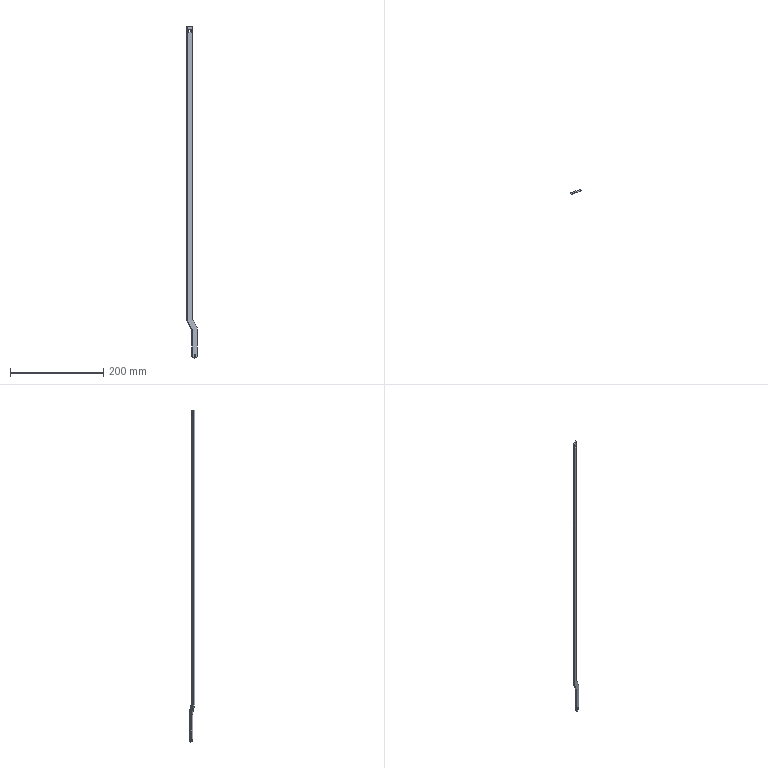Component | SolidWorks | RightDoorAssembly-1_LinkRodLock-1_LowerLinkRod1-1 | 1 solid | 21 faces | box 23.38 x 11.77 x 712 mm | volume 25523 mm3 | plane 13 | cylinder 8 | commonest cylinder face diameters 4.2 x2 12 x2 10 x2 34 x2
STEP:
#1=COLOUR_RGB('',0.7922,0.8196,0.9333);
#2=FILL_AREA_STYLE_COLOUR('',#1);
#3=FILL_AREA_STYLE('',(#2));
#4=SURFACE_STYLE_FILL_AREA(#3);
#5=SURFACE_SIDE_STYLE('',(#4));
#6=SURFACE_STYLE_USAGE(.BOTH.,#5);
#7=PRESENTATION_STYLE_ASSIGNMENT((#6));
#8=CARTESIAN_POINT('',(-12.447,16.163,3.811));
#9=VERTEX_POINT('',#8);
#10=CARTESIAN_POINT('',(-12.447,16.163,3.646));
#11=VERTEX_POINT('',#10);
#12=CARTESIAN_POINT('',(-12.447,16.163,3.728));
#13=DIRECTION('',(0.3744,-0.9273,0.));
#14=DIRECTION('',(0.,-0.,-1.));
#15=AXIS2_PLACEMENT_3D('',#12,#13,#14);
#16=CIRCLE('',#15,0.08268);
#17=EDGE_CURVE('',#9,#11,#16,.T.);
#18=ORIENTED_EDGE('',*,*,#17,.F.);
#19=CARTESIAN_POINT('',(-12.403,16.053,3.811));
#20=VERTEX_POINT('',#19);
#21=CARTESIAN_POINT('',(-12.447,16.163,3.811));
#22=DIRECTION('',(0.3744,-0.9273,0.));
#23=VECTOR('',#22,39.37);
#24=LINE('',#21,#23);
#25=EDGE_CURVE('',#9,#20,#24,.T.);
#26=ORIENTED_EDGE('',*,*,#25,.T.);
#27=CARTESIAN_POINT('',(-12.403,16.053,3.646));
#28=VERTEX_POINT('',#27);
#29=CARTESIAN_POINT('',(-12.403,16.053,3.728));
#30=DIRECTION('',(0.3744,-0.9273,0.));
#31=DIRECTION('',(0.,-0.,-1.));
#32=AXIS2_PLACEMENT_3D('',#29,#30,#31);
#33=CIRCLE('',#32,0.08268);
#34=EDGE_CURVE('',#20,#28,#33,.T.);
#35=ORIENTED_EDGE('',*,*,#34,.T.);
#36=CARTESIAN_POINT('',(-12.447,16.163,3.646));
#37=DIRECTION('',(0.3744,-0.9273,0.));
#38=VECTOR('',#37,39.37);
#39=LINE('',#36,#38);
#40=EDGE_CURVE('',#11,#28,#39,.T.);
#41=ORIENTED_EDGE('',*,*,#40,.F.);
#42=EDGE_LOOP('',(#18,#26,#35,#41));
#43=FACE_OUTER_BOUND('',#42,.T.);
#44=CARTESIAN_POINT('',(-12.447,16.163,3.728));
#45=DIRECTION('',(0.3744,-0.9273,0.));
#46=DIRECTION('',(0.,-0.,-1.));
#47=AXIS2_PLACEMENT_3D('',#44,#45,#46);
#48=CYLINDRICAL_SURFACE('',#47,0.08268);
#49=ADVANCED_FACE('',(#43),#48,.F.);
#50=CARTESIAN_POINT('',(-12.666,16.074,3.728));
#51=VERTEX_POINT('',#50);
#52=CARTESIAN_POINT('',(-12.447,16.163,3.492));
#53=VERTEX_POINT('',#52);
#54=CARTESIAN_POINT('',(-12.447,16.163,3.728));
#55=DIRECTION('',(0.3744,-0.9273,0.));
#56=DIRECTION('',(0.,-0.,-1.));
#57=AXIS2_PLACEMENT_3D('',#54,#55,#56);
#58=CIRCLE('',#57,0.2362);
#59=EDGE_CURVE('',#51,#53,#58,.T.);
#60=ORIENTED_EDGE('',*,*,#59,.T.);
#61=CARTESIAN_POINT('',(-12.403,16.053,3.492));
#62=VERTEX_POINT('',#61);
#63=CARTESIAN_POINT('',(-12.447,16.163,3.492));
#64=DIRECTION('',(0.3744,-0.9273,0.));
#65=VECTOR('',#64,39.37);
#66=LINE('',#63,#65);
#67=EDGE_CURVE('',#53,#62,#66,.T.);
#68=ORIENTED_EDGE('',*,*,#67,.T.);
#69=CARTESIAN_POINT('',(-12.622,15.965,3.728));
#70=VERTEX_POINT('',#69);
#71=CARTESIAN_POINT('',(-12.403,16.053,3.728));
#72=DIRECTION('',(0.3744,-0.9273,0.));
#73=DIRECTION('',(0.,-0.,-1.));
#74=AXIS2_PLACEMENT_3D('',#71,#72,#73);
#75=CIRCLE('',#74,0.2362);
#76=EDGE_CURVE('',#70,#62,#75,.T.);
#77=ORIENTED_EDGE('',*,*,#76,.F.);
#78=CARTESIAN_POINT('',(-12.666,16.074,3.728));
#79=DIRECTION('',(0.3744,-0.9273,0.));
#80=VECTOR('',#79,39.37);
#81=LINE('',#78,#80);
#82=EDGE_CURVE('',#51,#70,#81,.T.);
#83=ORIENTED_EDGE('',*,*,#82,.F.);
#84=EDGE_LOOP('',(#60,#68,#77,#83));
#85=FACE_OUTER_BOUND('',#84,.T.);
#86=CARTESIAN_POINT('',(-12.447,16.163,3.728));
#87=DIRECTION('',(0.3744,-0.9273,0.));
#88=DIRECTION('',(0.,-0.,-1.));
#89=AXIS2_PLACEMENT_3D('',#86,#87,#88);
#90=CYLINDRICAL_SURFACE('',#89,0.2362);
#91=ADVANCED_FACE('',(#85),#90,.T.);
#92=CARTESIAN_POINT('',(-13.06,15.788,31.524));
#93=VERTEX_POINT('',#92);
#94=CARTESIAN_POINT('',(-13.06,15.788,6.854));
#95=VERTEX_POINT('',#94);
#96=CARTESIAN_POINT('',(-13.06,15.788,31.524));
#97=DIRECTION('',(0.,-0.,-1.));
#98=VECTOR('',#97,39.37);
#99=LINE('',#96,#98);
#100=EDGE_CURVE('',#93,#95,#99,.T.);
#101=ORIENTED_EDGE('',*,*,#100,.F.);
#102=CARTESIAN_POINT('',(-13.104,15.897,31.524));
#103=VERTEX_POINT('',#102);
#104=CARTESIAN_POINT('',(-13.104,15.897,31.524));
#105=DIRECTION('',(0.3744,-0.9273,0.));
#106=VECTOR('',#105,39.37);
#107=LINE('',#104,#106);
#108=EDGE_CURVE('',#103,#93,#107,.T.);
#109=ORIENTED_EDGE('',*,*,#108,.F.);
#110=CARTESIAN_POINT('',(-13.104,15.897,6.854));
#111=VERTEX_POINT('',#110);
#112=CARTESIAN_POINT('',(-13.104,15.897,31.524));
#113=DIRECTION('',(0.,-0.,-1.));
#114=VECTOR('',#113,39.37);
#115=LINE('',#112,#114);
#116=EDGE_CURVE('',#103,#111,#115,.T.);
#117=ORIENTED_EDGE('',*,*,#116,.T.);
#118=CARTESIAN_POINT('',(-13.104,15.897,6.854));
#119=DIRECTION('',(0.3744,-0.9273,0.));
#120=VECTOR('',#119,39.37);
#121=LINE('',#118,#120);
#122=EDGE_CURVE('',#111,#95,#121,.T.);
#123=ORIENTED_EDGE('',*,*,#122,.T.);
#124=EDGE_LOOP('',(#101,#109,#117,#123));
#125=FACE_OUTER_BOUND('',#124,.T.);
#126=CARTESIAN_POINT('',(-13.104,15.897,31.524));
#127=DIRECTION('',(-0.9273,-0.3744,-0.));
#128=DIRECTION('',(0.,-0.,-1.));
#129=AXIS2_PLACEMENT_3D('',#126,#127,#128);
#130=PLANE('',#129);
#131=ADVANCED_FACE('',(#125),#130,.T.);
#132=CARTESIAN_POINT('',(-12.622,15.965,31.524));
#133=VERTEX_POINT('',#132);
#134=CARTESIAN_POINT('',(-12.622,15.965,31.524));
#135=DIRECTION('',(-0.9273,-0.3744,-0.));
#136=VECTOR('',#135,39.37);
#137=LINE('',#134,#136);
#138=EDGE_CURVE('',#133,#93,#137,.T.);
#139=ORIENTED_EDGE('',*,*,#138,.F.);
#140=CARTESIAN_POINT('',(-12.666,16.074,31.524));
#141=VERTEX_POINT('',#140);
#142=CARTESIAN_POINT('',(-12.666,16.074,31.524));
#143=DIRECTION('',(0.3744,-0.9273,0.));
#144=VECTOR('',#143,39.37);
#145=LINE('',#142,#144);
#146=EDGE_CURVE('',#141,#133,#145,.T.);
#147=ORIENTED_EDGE('',*,*,#146,.F.);
#148=CARTESIAN_POINT('',(-12.666,16.074,31.524));
#149=DIRECTION('',(-0.9273,-0.3744,-0.));
#150=VECTOR('',#149,39.37);
#151=LINE('',#148,#150);
#152=EDGE_CURVE('',#141,#103,#151,.T.);
#153=ORIENTED_EDGE('',*,*,#152,.T.);
#154=ORIENTED_EDGE('',*,*,#108,.T.);
#155=EDGE_LOOP('',(#139,#147,#153,#154));
#156=FACE_OUTER_BOUND('',#155,.T.);
#157=CARTESIAN_POINT('',(-12.666,16.074,31.524));
#158=DIRECTION('',(-0.,0.,1.));
#159=DIRECTION('',(0.3744,-0.9273,0.));
#160=AXIS2_PLACEMENT_3D('',#157,#158,#159);
#161=PLANE('',#160);
#162=ADVANCED_FACE('',(#156),#161,.T.);
#163=CARTESIAN_POINT('',(-12.622,15.965,6.854));
#164=VERTEX_POINT('',#163);
#165=CARTESIAN_POINT('',(-12.622,15.965,31.524));
#166=DIRECTION('',(-0.,0.,1.));
#167=VECTOR('',#166,39.37);
#168=LINE('',#165,#167);
#169=EDGE_CURVE('',#164,#133,#168,.T.);
#170=ORIENTED_EDGE('',*,*,#169,.F.);
#171=CARTESIAN_POINT('',(-12.666,16.074,6.854));
#172=VERTEX_POINT('',#171);
#173=CARTESIAN_POINT('',(-12.666,16.074,6.854));
#174=DIRECTION('',(0.3744,-0.9273,0.));
#175=VECTOR('',#174,39.37);
#176=LINE('',#173,#175);
#177=EDGE_CURVE('',#172,#164,#176,.T.);
#178=ORIENTED_EDGE('',*,*,#177,.F.);
#179=CARTESIAN_POINT('',(-12.666,16.074,31.524));
#180=DIRECTION('',(-0.,0.,1.));
#181=VECTOR('',#180,39.37);
#182=LINE('',#179,#181);
#183=EDGE_CURVE('',#172,#141,#182,.T.);
#184=ORIENTED_EDGE('',*,*,#183,.T.);
#185=ORIENTED_EDGE('',*,*,#146,.T.);
#186=EDGE_LOOP('',(#170,#178,#184,#185));
#187=FACE_OUTER_BOUND('',#186,.T.);
#188=CARTESIAN_POINT('',(-12.666,16.074,31.524));
#189=DIRECTION('',(0.9273,0.3744,0.));
#190=DIRECTION('',(-0.,0.,1.));
#191=AXIS2_PLACEMENT_3D('',#188,#189,#190);
#192=PLANE('',#191);
#193=ADVANCED_FACE('',(#187),#192,.T.);
#194=CARTESIAN_POINT('',(-12.597,15.975,6.755));
#195=VERTEX_POINT('',#194);
#196=CARTESIAN_POINT('',(-12.439,16.038,6.854));
#197=DIRECTION('',(-0.3744,0.9273,-0.));
#198=DIRECTION('',(0.,-0.,-1.));
#199=AXIS2_PLACEMENT_3D('',#196,#197,#198);
#200=CIRCLE('',#199,0.1969);
#201=EDGE_CURVE('',#195,#164,#200,.T.);
#202=ORIENTED_EDGE('',*,*,#201,.F.);
#203=CARTESIAN_POINT('',(-12.641,16.084,6.755));
#204=VERTEX_POINT('',#203);
#205=CARTESIAN_POINT('',(-12.641,16.084,6.755));
#206=DIRECTION('',(0.3744,-0.9273,0.));
#207=VECTOR('',#206,39.37);
#208=LINE('',#205,#207);
#209=EDGE_CURVE('',#204,#195,#208,.T.);
#210=ORIENTED_EDGE('',*,*,#209,.F.);
#211=CARTESIAN_POINT('',(-12.483,16.148,6.854));
#212=DIRECTION('',(-0.3744,0.9273,-0.));
#213=DIRECTION('',(0.,-0.,-1.));
#214=AXIS2_PLACEMENT_3D('',#211,#212,#213);
#215=CIRCLE('',#214,0.1969);
#216=EDGE_CURVE('',#204,#172,#215,.T.);
#217=ORIENTED_EDGE('',*,*,#216,.T.);
#218=ORIENTED_EDGE('',*,*,#177,.T.);
#219=EDGE_LOOP('',(#202,#210,#217,#218));
#220=FACE_OUTER_BOUND('',#219,.T.);
#221=CARTESIAN_POINT('',(-12.483,16.148,6.854));
#222=DIRECTION('',(0.3744,-0.9273,0.));
#223=DIRECTION('',(0.,-0.,-1.));
#224=AXIS2_PLACEMENT_3D('',#221,#222,#223);
#225=CYLINDRICAL_SURFACE('',#224,0.1969);
#226=ADVANCED_FACE('',(#220),#225,.F.);
#227=CARTESIAN_POINT('',(-12.267,16.108,6.138));
#228=VERTEX_POINT('',#227);
#229=CARTESIAN_POINT('',(-12.267,16.108,6.138));
#230=DIRECTION('',(-0.4636,-0.1872,0.866));
#231=VECTOR('',#230,39.37);
#232=LINE('',#229,#231);
#233=EDGE_CURVE('',#228,#195,#232,.T.);
#234=ORIENTED_EDGE('',*,*,#233,.F.);
#235=CARTESIAN_POINT('',(-12.311,16.218,6.138));
#236=VERTEX_POINT('',#235);
#237=CARTESIAN_POINT('',(-12.311,16.218,6.138));
#238=DIRECTION('',(0.3744,-0.9273,0.));
#239=VECTOR('',#238,39.37);
#240=LINE('',#237,#239);
#241=EDGE_CURVE('',#236,#228,#240,.T.);
#242=ORIENTED_EDGE('',*,*,#241,.F.);
#243=CARTESIAN_POINT('',(-12.311,16.218,6.138));
#244=DIRECTION('',(-0.4636,-0.1872,0.866));
#245=VECTOR('',#244,39.37);
#246=LINE('',#243,#245);
#247=EDGE_CURVE('',#236,#204,#246,.T.);
#248=ORIENTED_EDGE('',*,*,#247,.T.);
#249=ORIENTED_EDGE('',*,*,#209,.T.);
#250=EDGE_LOOP('',(#234,#242,#248,#249));
#251=FACE_OUTER_BOUND('',#250,.T.);
#252=CARTESIAN_POINT('',(-12.311,16.218,6.138));
#253=DIRECTION('',(0.803,0.3242,0.5));
#254=DIRECTION('',(-0.4636,-0.1872,0.866));
#255=AXIS2_PLACEMENT_3D('',#252,#253,#254);
#256=PLANE('',#255);
#257=ADVANCED_FACE('',(#251),#256,.T.);
#258=CARTESIAN_POINT('',(-12.184,16.142,5.803));
#259=VERTEX_POINT('',#258);
#260=CARTESIAN_POINT('',(-12.804,15.891,5.803));
#261=DIRECTION('',(0.3744,-0.9273,0.));
#262=DIRECTION('',(0.,-0.,-1.));
#263=AXIS2_PLACEMENT_3D('',#260,#261,#262);
#264=CIRCLE('',#263,0.6693);
#265=EDGE_CURVE('',#259,#228,#264,.T.);
#266=ORIENTED_EDGE('',*,*,#265,.F.);
#267=CARTESIAN_POINT('',(-12.228,16.251,5.803));
#268=VERTEX_POINT('',#267);
#269=CARTESIAN_POINT('',(-12.228,16.251,5.803));
#270=DIRECTION('',(0.3744,-0.9273,0.));
#271=VECTOR('',#270,39.37);
#272=LINE('',#269,#271);
#273=EDGE_CURVE('',#268,#259,#272,.T.);
#274=ORIENTED_EDGE('',*,*,#273,.F.);
#275=CARTESIAN_POINT('',(-12.848,16.001,5.803));
#276=DIRECTION('',(0.3744,-0.9273,0.));
#277=DIRECTION('',(0.,-0.,-1.));
#278=AXIS2_PLACEMENT_3D('',#275,#276,#277);
#279=CIRCLE('',#278,0.6693);
#280=EDGE_CURVE('',#268,#236,#279,.T.);
#281=ORIENTED_EDGE('',*,*,#280,.T.);
#282=ORIENTED_EDGE('',*,*,#241,.T.);
#283=EDGE_LOOP('',(#266,#274,#281,#282));
#284=FACE_OUTER_BOUND('',#283,.T.);
#285=CARTESIAN_POINT('',(-12.848,16.001,5.803));
#286=DIRECTION('',(0.3744,-0.9273,0.));
#287=DIRECTION('',(0.,-0.,-1.));
#288=AXIS2_PLACEMENT_3D('',#285,#286,#287);
#289=CYLINDRICAL_SURFACE('',#288,0.6693);
#290=ADVANCED_FACE('',(#284),#289,.T.);
#291=CARTESIAN_POINT('',(-12.184,16.142,3.728));
#292=VERTEX_POINT('',#291);
#293=CARTESIAN_POINT('',(-12.184,16.142,5.803));
#294=DIRECTION('',(-0.,0.,1.));
#295=VECTOR('',#294,39.37);
#296=LINE('',#293,#295);
#297=EDGE_CURVE('',#292,#259,#296,.T.);
#298=ORIENTED_EDGE('',*,*,#297,.F.);
#299=CARTESIAN_POINT('',(-12.228,16.251,3.728));
#300=VERTEX_POINT('',#299);
#301=CARTESIAN_POINT('',(-12.228,16.251,3.728));
#302=DIRECTION('',(0.3744,-0.9273,0.));
#303=VECTOR('',#302,39.37);
#304=LINE('',#301,#303);
#305=EDGE_CURVE('',#300,#292,#304,.T.);
#306=ORIENTED_EDGE('',*,*,#305,.F.);
#307=CARTESIAN_POINT('',(-12.228,16.251,5.803));
#308=DIRECTION('',(-0.,0.,1.));
#309=VECTOR('',#308,39.37);
#310=LINE('',#307,#309);
#311=EDGE_CURVE('',#300,#268,#310,.T.);
#312=ORIENTED_EDGE('',*,*,#311,.T.);
#313=ORIENTED_EDGE('',*,*,#273,.T.);
#314=EDGE_LOOP('',(#298,#306,#312,#313));
#315=FACE_OUTER_BOUND('',#314,.T.);
#316=CARTESIAN_POINT('',(-12.228,16.251,5.803));
#317=DIRECTION('',(0.9273,0.3744,-0.));
#318=DIRECTION('',(-0.,0.,1.));
#319=AXIS2_PLACEMENT_3D('',#316,#317,#318);
#320=PLANE('',#319);
#321=ADVANCED_FACE('',(#315),#320,.T.);
#322=ORIENTED_EDGE('',*,*,#67,.F.);
#323=CARTESIAN_POINT('',(-12.447,16.163,3.728));
#324=DIRECTION('',(0.3744,-0.9273,0.));
#325=DIRECTION('',(0.,-0.,-1.));
#326=AXIS2_PLACEMENT_3D('',#323,#324,#325);
#327=CIRCLE('',#326,0.2362);
#328=EDGE_CURVE('',#53,#300,#327,.T.);
#329=ORIENTED_EDGE('',*,*,#328,.T.);
#330=ORIENTED_EDGE('',*,*,#305,.T.);
#331=CARTESIAN_POINT('',(-12.403,16.053,3.728));
#332=DIRECTION('',(0.3744,-0.9273,0.));
#333=DIRECTION('',(0.,-0.,-1.));
#334=AXIS2_PLACEMENT_3D('',#331,#332,#333);
#335=CIRCLE('',#334,0.2362);
#336=EDGE_CURVE('',#62,#292,#335,.T.);
#337=ORIENTED_EDGE('',*,*,#336,.F.);
#338=EDGE_LOOP('',(#322,#329,#330,#337));
#339=FACE_OUTER_BOUND('',#338,.T.);
#340=CARTESIAN_POINT('',(-12.447,16.163,3.728));
#341=DIRECTION('',(0.3744,-0.9273,0.));
#342=DIRECTION('',(0.,-0.,-1.));
#343=AXIS2_PLACEMENT_3D('',#340,#341,#342);
#344=CYLINDRICAL_SURFACE('',#343,0.2362);
#345=ADVANCED_FACE('',(#339),#344,.T.);
#346=CARTESIAN_POINT('',(-12.622,15.965,5.803));
#347=VERTEX_POINT('',#346);
#348=CARTESIAN_POINT('',(-12.622,15.965,5.803));
#349=DIRECTION('',(0.,-0.,-1.));
#350=VECTOR('',#349,39.37);
#351=LINE('',#348,#350);
#352=EDGE_CURVE('',#347,#70,#351,.T.);
#353=ORIENTED_EDGE('',*,*,#352,.F.);
#354=CARTESIAN_POINT('',(-12.666,16.074,5.803));
#355=VERTEX_POINT('',#354);
#356=CARTESIAN_POINT('',(-12.666,16.074,5.803));
#357=DIRECTION('',(0.3744,-0.9273,0.));
#358=VECTOR('',#357,39.37);
#359=LINE('',#356,#358);
#360=EDGE_CURVE('',#355,#347,#359,.T.);
#361=ORIENTED_EDGE('',*,*,#360,.F.);
#362=CARTESIAN_POINT('',(-12.666,16.074,5.803));
#363=DIRECTION('',(0.,-0.,-1.));
#364=VECTOR('',#363,39.37);
#365=LINE('',#362,#364);
#366=EDGE_CURVE('',#355,#51,#365,.T.);
#367=ORIENTED_EDGE('',*,*,#366,.T.);
#368=ORIENTED_EDGE('',*,*,#82,.T.);
#369=EDGE_LOOP('',(#353,#361,#367,#368));
#370=FACE_OUTER_BOUND('',#369,.T.);
#371=CARTESIAN_POINT('',(-12.666,16.074,5.803));
#372=DIRECTION('',(-0.9273,-0.3744,-0.));
#373=DIRECTION('',(0.,-0.,-1.));
#374=AXIS2_PLACEMENT_3D('',#371,#372,#373);
#375=PLANE('',#374);
#376=ADVANCED_FACE('',(#370),#375,.T.);
#377=CARTESIAN_POINT('',(-12.646,15.955,5.902));
#378=VERTEX_POINT('',#377);
#379=CARTESIAN_POINT('',(-12.804,15.891,5.803));
#380=DIRECTION('',(-0.3744,0.9273,-0.));
#381=DIRECTION('',(0.,-0.,-1.));
#382=AXIS2_PLACEMENT_3D('',#379,#380,#381);
#383=CIRCLE('',#382,0.1969);
#384=EDGE_CURVE('',#378,#347,#383,.T.);
#385=ORIENTED_EDGE('',*,*,#384,.F.);
#386=CARTESIAN_POINT('',(-12.69,16.064,5.902));
#387=VERTEX_POINT('',#386);
#388=CARTESIAN_POINT('',(-12.69,16.064,5.902));
#389=DIRECTION('',(0.3744,-0.9273,0.));
#390=VECTOR('',#389,39.37);
#391=LINE('',#388,#390);
#392=EDGE_CURVE('',#387,#378,#391,.T.);
#393=ORIENTED_EDGE('',*,*,#392,.F.);
#394=CARTESIAN_POINT('',(-12.848,16.001,5.803));
#395=DIRECTION('',(-0.3744,0.9273,-0.));
#396=DIRECTION('',(0.,-0.,-1.));
#397=AXIS2_PLACEMENT_3D('',#394,#395,#396);
#398=CIRCLE('',#397,0.1969);
#399=EDGE_CURVE('',#387,#355,#398,.T.);
#400=ORIENTED_EDGE('',*,*,#399,.T.);
#401=ORIENTED_EDGE('',*,*,#360,.T.);
#402=EDGE_LOOP('',(#385,#393,#400,#401));
#403=FACE_OUTER_BOUND('',#402,.T.);
#404=CARTESIAN_POINT('',(-12.848,16.001,5.803));
#405=DIRECTION('',(0.3744,-0.9273,0.));
#406=DIRECTION('',(0.,-0.,-1.));
#407=AXIS2_PLACEMENT_3D('',#404,#405,#406);
#408=CYLINDRICAL_SURFACE('',#407,0.1969);
#409=ADVANCED_FACE('',(#403),#408,.F.);
#410=CARTESIAN_POINT('',(-12.977,15.821,6.519));
#411=VERTEX_POINT('',#410);
#412=CARTESIAN_POINT('',(-12.646,15.955,5.902));
#413=DIRECTION('',(0.4636,0.1872,-0.866));
#414=VECTOR('',#413,39.37);
#415=LINE('',#412,#414);
#416=EDGE_CURVE('',#411,#378,#415,.T.);
#417=ORIENTED_EDGE('',*,*,#416,.F.);
#418=CARTESIAN_POINT('',(-13.021,15.931,6.519));
#419=VERTEX_POINT('',#418);
#420=CARTESIAN_POINT('',(-13.021,15.931,6.519));
#421=DIRECTION('',(0.3744,-0.9273,0.));
#422=VECTOR('',#421,39.37);
#423=LINE('',#420,#422);
#424=EDGE_CURVE('',#419,#411,#423,.T.);
#425=ORIENTED_EDGE('',*,*,#424,.F.);
#426=CARTESIAN_POINT('',(-12.69,16.064,5.902));
#427=DIRECTION('',(0.4636,0.1872,-0.866));
#428=VECTOR('',#427,39.37);
#429=LINE('',#426,#428);
#430=EDGE_CURVE('',#419,#387,#429,.T.);
#431=ORIENTED_EDGE('',*,*,#430,.T.);
#432=ORIENTED_EDGE('',*,*,#392,.T.);
#433=EDGE_LOOP('',(#417,#425,#431,#432));
#434=FACE_OUTER_BOUND('',#433,.T.);
#435=CARTESIAN_POINT('',(-12.69,16.064,5.902));
#436=DIRECTION('',(-0.803,-0.3242,-0.5));
#437=DIRECTION('',(0.4636,0.1872,-0.866));
#438=AXIS2_PLACEMENT_3D('',#435,#436,#437);
#439=PLANE('',#438);
#440=ADVANCED_FACE('',(#434),#439,.T.);
#441=CARTESIAN_POINT('',(-12.439,16.038,6.854));
#442=DIRECTION('',(0.3744,-0.9273,0.));
#443=DIRECTION('',(0.,-0.,-1.));
#444=AXIS2_PLACEMENT_3D('',#441,#442,#443);
#445=CIRCLE('',#444,0.6693);
#446=EDGE_CURVE('',#95,#411,#445,.T.);
#447=ORIENTED_EDGE('',*,*,#446,.F.);
#448=ORIENTED_EDGE('',*,*,#122,.F.);
#449=CARTESIAN_POINT('',(-12.483,16.148,6.854));
#450=DIRECTION('',(0.3744,-0.9273,0.));
#451=DIRECTION('',(0.,-0.,-1.));
#452=AXIS2_PLACEMENT_3D('',#449,#450,#451);
#453=CIRCLE('',#452,0.6693);
#454=EDGE_CURVE('',#111,#419,#453,.T.);
#455=ORIENTED_EDGE('',*,*,#454,.T.);
#456=ORIENTED_EDGE('',*,*,#424,.T.);
#457=EDGE_LOOP('',(#447,#448,#455,#456));
#458=FACE_OUTER_BOUND('',#457,.T.);
#459=CARTESIAN_POINT('',(-12.483,16.148,6.854));
#460=DIRECTION('',(0.3744,-0.9273,0.));
#461=DIRECTION('',(0.,-0.,-1.));
#462=AXIS2_PLACEMENT_3D('',#459,#460,#461);
#463=CYLINDRICAL_SURFACE('',#462,0.6693);
#464=ADVANCED_FACE('',(#458),#463,.T.);
#465=CARTESIAN_POINT('',(-12.447,16.163,3.728));
#466=DIRECTION('',(0.3744,-0.9273,0.));
#467=DIRECTION('',(0.,-0.,-1.));
#468=AXIS2_PLACEMENT_3D('',#465,#466,#467);
#469=CIRCLE('',#468,0.08268);
#470=EDGE_CURVE('',#11,#9,#469,.T.);
#471=ORIENTED_EDGE('',*,*,#470,.T.);
#472=ORIENTED_EDGE('',*,*,#17,.T.);
#473=EDGE_LOOP('',(#471,#472));
#474=FACE_BOUND('',#473,.T.);
#475=CARTESIAN_POINT('',(-13.004,15.938,31.002));
#476=VERTEX_POINT('',#475);
#477=CARTESIAN_POINT('',(-12.766,16.034,31.002));
#478=VERTEX_POINT('',#477);
#479=CARTESIAN_POINT('',(-12.766,16.034,31.002));
#480=DIRECTION('',(0.9273,0.3744,0.));
#481=VECTOR('',#480,39.37);
#482=LINE('',#479,#481);
#483=EDGE_CURVE('',#476,#478,#482,.T.);
#484=ORIENTED_EDGE('',*,*,#483,.T.);
#485=CARTESIAN_POINT('',(-12.766,16.034,31.258));
#486=VERTEX_POINT('',#485);
#487=CARTESIAN_POINT('',(-12.766,16.034,31.258));
#488=DIRECTION('',(-0.,0.,1.));
#489=VECTOR('',#488,39.37);
#490=LINE('',#487,#489);
#491=EDGE_CURVE('',#478,#486,#490,.T.);
#492=ORIENTED_EDGE('',*,*,#491,.T.);
#493=CARTESIAN_POINT('',(-13.004,15.938,31.258));
#494=VERTEX_POINT('',#493);
#495=CARTESIAN_POINT('',(-13.004,15.938,31.258));
#496=DIRECTION('',(-0.9273,-0.3744,-0.));
#497=VECTOR('',#496,39.37);
#498=LINE('',#495,#497);
#499=EDGE_CURVE('',#486,#494,#498,.T.);
#500=ORIENTED_EDGE('',*,*,#499,.T.);
#501=CARTESIAN_POINT('',(-13.004,15.938,31.002));
#502=DIRECTION('',(0.,-0.,-1.));
#503=VECTOR('',#502,39.37);
#504=LINE('',#501,#503);
#505=EDGE_CURVE('',#494,#476,#504,.T.);
#506=ORIENTED_EDGE('',*,*,#505,.T.);
#507=EDGE_LOOP('',(#484,#492,#500,#506));
#508=FACE_BOUND('',#507,.T.);
#509=ORIENTED_EDGE('',*,*,#116,.F.);
#510=ORIENTED_EDGE('',*,*,#152,.F.);
#511=ORIENTED_EDGE('',*,*,#183,.F.);
#512=ORIENTED_EDGE('',*,*,#216,.F.);
#513=ORIENTED_EDGE('',*,*,#247,.F.);
#514=ORIENTED_EDGE('',*,*,#280,.F.);
#515=ORIENTED_EDGE('',*,*,#311,.F.);
#516=ORIENTED_EDGE('',*,*,#328,.F.);
#517=ORIENTED_EDGE('',*,*,#59,.F.);
#518=ORIENTED_EDGE('',*,*,#366,.F.);
#519=ORIENTED_EDGE('',*,*,#399,.F.);
#520=ORIENTED_EDGE('',*,*,#430,.F.);
#521=ORIENTED_EDGE('',*,*,#454,.F.);
#522=EDGE_LOOP('',(#509,#510,#511,#512,#513,#514,#515,#516,#517,#518,#519,#520,#521));
#523=FACE_OUTER_BOUND('',#522,.T.);
#524=CARTESIAN_POINT('',(-12.483,16.148,6.854));
#525=DIRECTION('',(0.3744,-0.9273,0.));
#526=DIRECTION('',(0.,-0.,-1.));
#527=AXIS2_PLACEMENT_3D('',#524,#525,#526);
#528=PLANE('',#527);
#529=ADVANCED_FACE('',(#474,#508,#523),#528,.F.);
#530=CARTESIAN_POINT('',(-12.403,16.053,3.728));
#531=DIRECTION('',(0.3744,-0.9273,0.));
#532=DIRECTION('',(0.,-0.,-1.));
#533=AXIS2_PLACEMENT_3D('',#530,#531,#532);
#534=CIRCLE('',#533,0.08268);
#535=EDGE_CURVE('',#28,#20,#534,.T.);
#536=ORIENTED_EDGE('',*,*,#535,.F.);
#537=ORIENTED_EDGE('',*,*,#34,.F.);
#538=EDGE_LOOP('',(#536,#537));
#539=FACE_BOUND('',#538,.T.);
#540=CARTESIAN_POINT('',(-12.722,15.924,31.002));
#541=VERTEX_POINT('',#540);
#542=CARTESIAN_POINT('',(-12.722,15.924,31.258));
#543=VERTEX_POINT('',#542);
#544=CARTESIAN_POINT('',(-12.722,15.924,31.258));
#545=DIRECTION('',(-0.,0.,1.));
#546=VECTOR('',#545,39.37);
#547=LINE('',#544,#546);
#548=EDGE_CURVE('',#541,#543,#547,.T.);
#549=ORIENTED_EDGE('',*,*,#548,.F.);
#550=CARTESIAN_POINT('',(-12.959,15.828,31.002));
#551=VERTEX_POINT('',#550);
#552=CARTESIAN_POINT('',(-12.722,15.924,31.002));
#553=DIRECTION('',(0.9273,0.3744,0.));
#554=VECTOR('',#553,39.37);
#555=LINE('',#552,#554);
#556=EDGE_CURVE('',#551,#541,#555,.T.);
#557=ORIENTED_EDGE('',*,*,#556,.F.);
#558=CARTESIAN_POINT('',(-12.959,15.828,31.258));
#559=VERTEX_POINT('',#558);
#560=CARTESIAN_POINT('',(-12.959,15.828,31.002));
#561=DIRECTION('',(0.,-0.,-1.));
#562=VECTOR('',#561,39.37);
#563=LINE('',#560,#562);
#564=EDGE_CURVE('',#559,#551,#563,.T.);
#565=ORIENTED_EDGE('',*,*,#564,.F.);
#566=CARTESIAN_POINT('',(-12.959,15.828,31.258));
#567=DIRECTION('',(-0.9273,-0.3744,-0.));
#568=VECTOR('',#567,39.37);
#569=LINE('',#566,#568);
#570=EDGE_CURVE('',#543,#559,#569,.T.);
#571=ORIENTED_EDGE('',*,*,#570,.F.);
#572=EDGE_LOOP('',(#549,#557,#565,#571));
#573=FACE_BOUND('',#572,.T.);
#574=ORIENTED_EDGE('',*,*,#100,.T.);
#575=ORIENTED_EDGE('',*,*,#446,.T.);
#576=ORIENTED_EDGE('',*,*,#416,.T.);
#577=ORIENTED_EDGE('',*,*,#384,.T.);
#578=ORIENTED_EDGE('',*,*,#352,.T.);
#579=ORIENTED_EDGE('',*,*,#76,.T.);
#580=ORIENTED_EDGE('',*,*,#336,.T.);
#581=ORIENTED_EDGE('',*,*,#297,.T.);
#582=ORIENTED_EDGE('',*,*,#265,.T.);
#583=ORIENTED_EDGE('',*,*,#233,.T.);
#584=ORIENTED_EDGE('',*,*,#201,.T.);
#585=ORIENTED_EDGE('',*,*,#169,.T.);
#586=ORIENTED_EDGE('',*,*,#138,.T.);
#587=EDGE_LOOP('',(#574,#575,#576,#577,#578,#579,#580,#581,#582,#583,#584,#585,#586));
#588=FACE_OUTER_BOUND('',#587,.T.);
#589=CARTESIAN_POINT('',(-12.439,16.038,6.854));
#590=DIRECTION('',(0.3744,-0.9273,0.));
#591=DIRECTION('',(0.,-0.,-1.));
#592=AXIS2_PLACEMENT_3D('',#589,#590,#591);
#593=PLANE('',#592);
#594=ADVANCED_FACE('',(#539,#573,#588),#593,.T.);
#595=ORIENTED_EDGE('',*,*,#548,.T.);
#596=CARTESIAN_POINT('',(-12.766,16.034,31.258));
#597=DIRECTION('',(0.3744,-0.9273,0.));
#598=VECTOR('',#597,39.37);
#599=LINE('',#596,#598);
#600=EDGE_CURVE('',#486,#543,#599,.T.);
#601=ORIENTED_EDGE('',*,*,#600,.F.);
#602=ORIENTED_EDGE('',*,*,#491,.F.);
#603=CARTESIAN_POINT('',(-12.766,16.034,31.002));
#604=DIRECTION('',(0.3744,-0.9273,0.));
#605=VECTOR('',#604,39.37);
#606=LINE('',#603,#605);
#607=EDGE_CURVE('',#478,#541,#606,.T.);
#608=ORIENTED_EDGE('',*,*,#607,.T.);
#609=EDGE_LOOP('',(#595,#601,#602,#608));
#610=FACE_OUTER_BOUND('',#609,.T.);
#611=CARTESIAN_POINT('',(-12.766,16.034,31.258));
#612=DIRECTION('',(0.9273,0.3744,0.));
#613=DIRECTION('',(0.3744,-0.9273,0.));
#614=AXIS2_PLACEMENT_3D('',#611,#612,#613);
#615=PLANE('',#614);
#616=ADVANCED_FACE('',(#610),#615,.F.);
#617=ORIENTED_EDGE('',*,*,#556,.T.);
#618=ORIENTED_EDGE('',*,*,#607,.F.);
#619=ORIENTED_EDGE('',*,*,#483,.F.);
#620=CARTESIAN_POINT('',(-13.004,15.938,31.002));
#621=DIRECTION('',(0.3744,-0.9273,0.));
#622=VECTOR('',#621,39.37);
#623=LINE('',#620,#622);
#624=EDGE_CURVE('',#476,#551,#623,.T.);
#625=ORIENTED_EDGE('',*,*,#624,.T.);
#626=EDGE_LOOP('',(#617,#618,#619,#625));
#627=FACE_OUTER_BOUND('',#626,.T.);
#628=CARTESIAN_POINT('',(-12.766,16.034,31.002));
#629=DIRECTION('',(0.,-0.,-1.));
#630=DIRECTION('',(-0.3744,0.9273,-0.));
#631=AXIS2_PLACEMENT_3D('',#628,#629,#630);
#632=PLANE('',#631);
#633=ADVANCED_FACE('',(#627),#632,.F.);
#634=ORIENTED_EDGE('',*,*,#564,.T.);
#635=ORIENTED_EDGE('',*,*,#624,.F.);
#636=ORIENTED_EDGE('',*,*,#505,.F.);
#637=CARTESIAN_POINT('',(-13.004,15.938,31.258));
#638=DIRECTION('',(0.3744,-0.9273,0.));
#639=VECTOR('',#638,39.37);
#640=LINE('',#637,#639);
#641=EDGE_CURVE('',#494,#559,#640,.T.);
#642=ORIENTED_EDGE('',*,*,#641,.T.);
#643=EDGE_LOOP('',(#634,#635,#636,#642));
#644=FACE_OUTER_BOUND('',#643,.T.);
#645=CARTESIAN_POINT('',(-13.004,15.938,31.002));
#646=DIRECTION('',(-0.9273,-0.3744,-0.));
#647=DIRECTION('',(0.,-0.,-1.));
#648=AXIS2_PLACEMENT_3D('',#645,#646,#647);
#649=PLANE('',#648);
#650=ADVANCED_FACE('',(#644),#649,.F.);
#651=ORIENTED_EDGE('',*,*,#570,.T.);
#652=ORIENTED_EDGE('',*,*,#641,.F.);
#653=ORIENTED_EDGE('',*,*,#499,.F.);
#654=ORIENTED_EDGE('',*,*,#600,.T.);
#655=EDGE_LOOP('',(#651,#652,#653,#654));
#656=FACE_OUTER_BOUND('',#655,.T.);
#657=CARTESIAN_POINT('',(-13.004,15.938,31.258));
#658=DIRECTION('',(-0.,0.,1.));
#659=DIRECTION('',(0.3744,-0.9273,0.));
#660=AXIS2_PLACEMENT_3D('',#657,#658,#659);
#661=PLANE('',#660);
#662=ADVANCED_FACE('',(#656),#661,.F.);
#663=ORIENTED_EDGE('',*,*,#25,.F.);
#664=ORIENTED_EDGE('',*,*,#470,.F.);
#665=ORIENTED_EDGE('',*,*,#40,.T.);
#666=ORIENTED_EDGE('',*,*,#535,.T.);
#667=EDGE_LOOP('',(#663,#664,#665,#666));
#668=FACE_OUTER_BOUND('',#667,.T.);
#669=CARTESIAN_POINT('',(-12.447,16.163,3.728));
#670=DIRECTION('',(0.3744,-0.9273,0.));
#671=DIRECTION('',(0.,-0.,-1.));
#672=AXIS2_PLACEMENT_3D('',#669,#670,#671);
#673=CYLINDRICAL_SURFACE('',#672,0.08268);
#674=ADVANCED_FACE('',(#668),#673,.F.);
#675=CLOSED_SHELL('',(#49,#91,#131,#162,#193,#226,#257,#290,#321,#345,#376,#409,#440,#464,#529,#594,#616,#633,#650,#662,#674));
#676=MANIFOLD_SOLID_BREP('',#675);
#677=STYLED_ITEM('',(#7),#676);
#678=(LENGTH_UNIT()NAMED_UNIT(*)SI_UNIT($,.METRE.));
#679=LENGTH_MEASURE_WITH_UNIT(LENGTH_MEASURE(0.0254),#678);
#680=DIMENSIONAL_EXPONENTS(1.,0.,0.,0.,0.,0.,0.);
#681=(CONVERSION_BASED_UNIT('',#679)LENGTH_UNIT()NAMED_UNIT(#680));
#682=UNCERTAINTY_MEASURE_WITH_UNIT(LENGTH_MEASURE(0.00001),#681,'','');
#683=(NAMED_UNIT(*)PLANE_ANGLE_UNIT()SI_UNIT($,.RADIAN.));
#684=(NAMED_UNIT(*)SI_UNIT($,.STERADIAN.)SOLID_ANGLE_UNIT());
#685=(GEOMETRIC_REPRESENTATION_CONTEXT(3)GLOBAL_UNCERTAINTY_ASSIGNED_CONTEXT((#682))GLOBAL_UNIT_ASSIGNED_CONTEXT((#681,#683,#684))REPRESENTATION_CONTEXT('',''));
#686=MECHANICAL_DESIGN_GEOMETRIC_PRESENTATION_REPRESENTATION('',(#677),#685);
#687=PRESENTATION_LAYER_ASSIGNMENT('','',(#677));
#688=CARTESIAN_POINT('',(0.,0.,0.));
#689=DIRECTION('',(0.,0.,1.));
#690=DIRECTION('',(1.,0.,0.));
#691=AXIS2_PLACEMENT_3D('',#688,#689,#690);
#692=(LENGTH_UNIT()NAMED_UNIT(*)SI_UNIT($,.METRE.));
#693=LENGTH_MEASURE_WITH_UNIT(LENGTH_MEASURE(0.0254),#692);
#694=DIMENSIONAL_EXPONENTS(1.,0.,0.,0.,0.,0.,0.);
#695=(CONVERSION_BASED_UNIT('',#693)LENGTH_UNIT()NAMED_UNIT(#694));
#696=UNCERTAINTY_MEASURE_WITH_UNIT(LENGTH_MEASURE(0.00001),#695,'','');
#697=(NAMED_UNIT(*)PLANE_ANGLE_UNIT()SI_UNIT($,.RADIAN.));
#698=(NAMED_UNIT(*)SI_UNIT($,.STERADIAN.)SOLID_ANGLE_UNIT());
#699=(GEOMETRIC_REPRESENTATION_CONTEXT(3)GLOBAL_UNCERTAINTY_ASSIGNED_CONTEXT((#696))GLOBAL_UNIT_ASSIGNED_CONTEXT((#695,#697,#698))REPRESENTATION_CONTEXT('',''));
#700=ADVANCED_BREP_SHAPE_REPRESENTATION('',(#676,#691),#699);